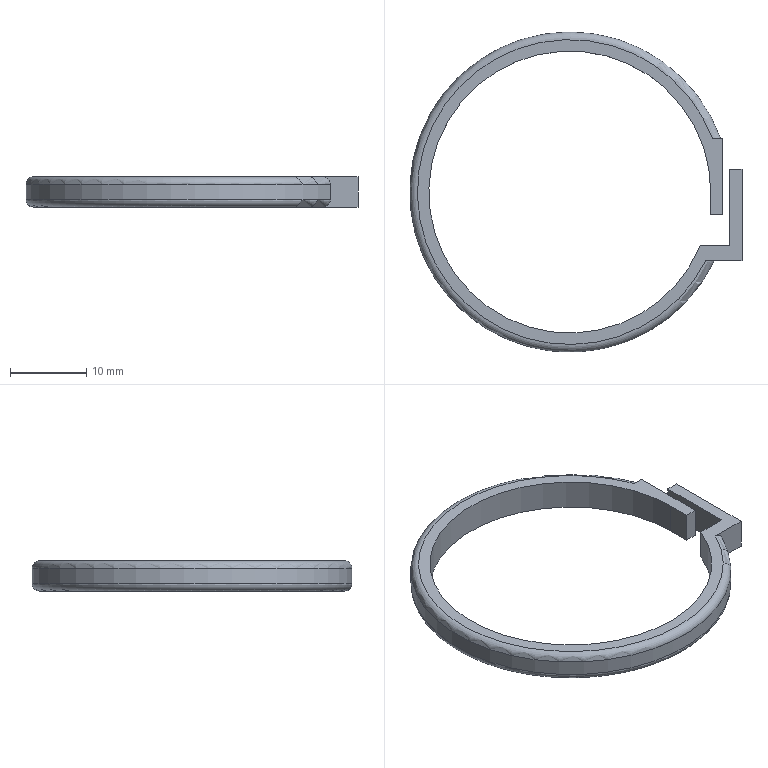Component | NX | CLAMP | 1 solid | 15 faces | volume 1215 mm3 | plane 11 | cylinder 2 | torus 2 | commonest cylinder face diameters 37 x1 42 x1